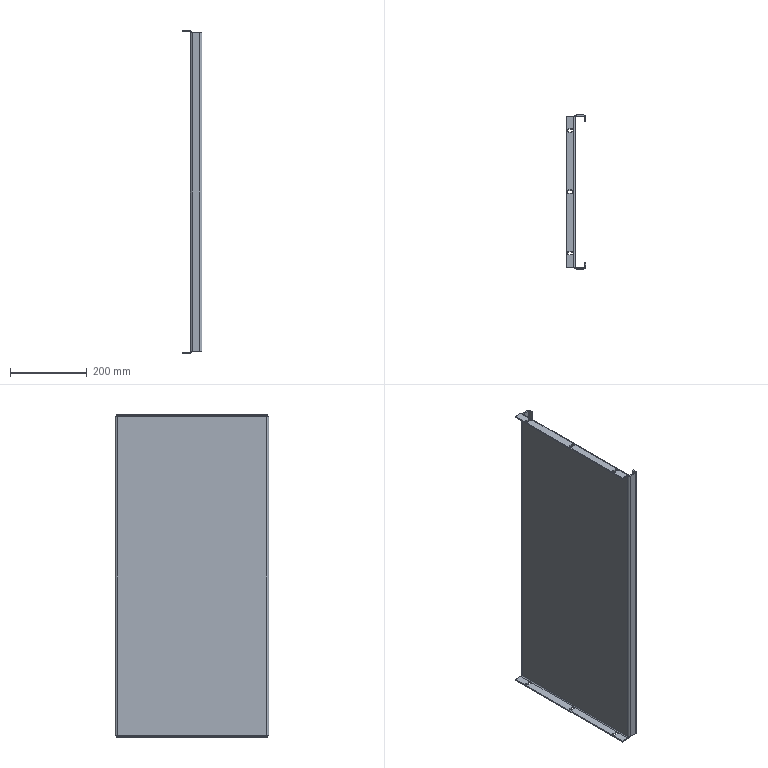Component | SolidWorks | CapacitorMountingPlateF6-00-1 | 1 solid | 88 faces | volume 1233206 mm3 | plane 58 | cylinder 30 | commonest cylinder face diameters 9 x18 11 x6 5 x6